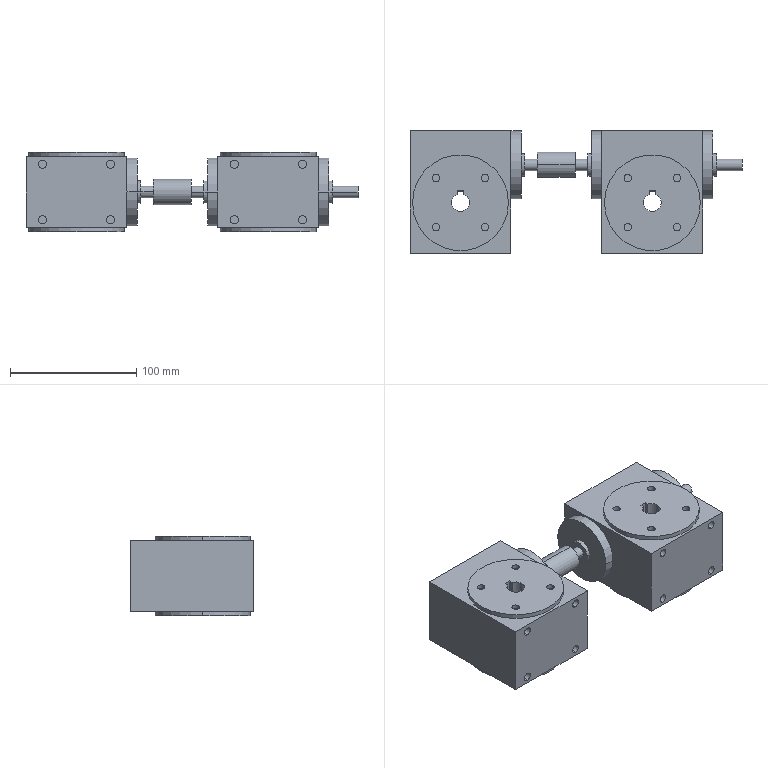Component | SolidWorks | DoubleFilmTransport-1_WormGearReducerNRV30-10-L+R-1 | 1 solid | 179 faces | volume 972844 mm3 | cylinder 110 | plane 69 | commonest cylinder face diameters 6 x32 6.5 x32 5 x12 76 x8 14 x6 9 x6 18 x6 54 x6